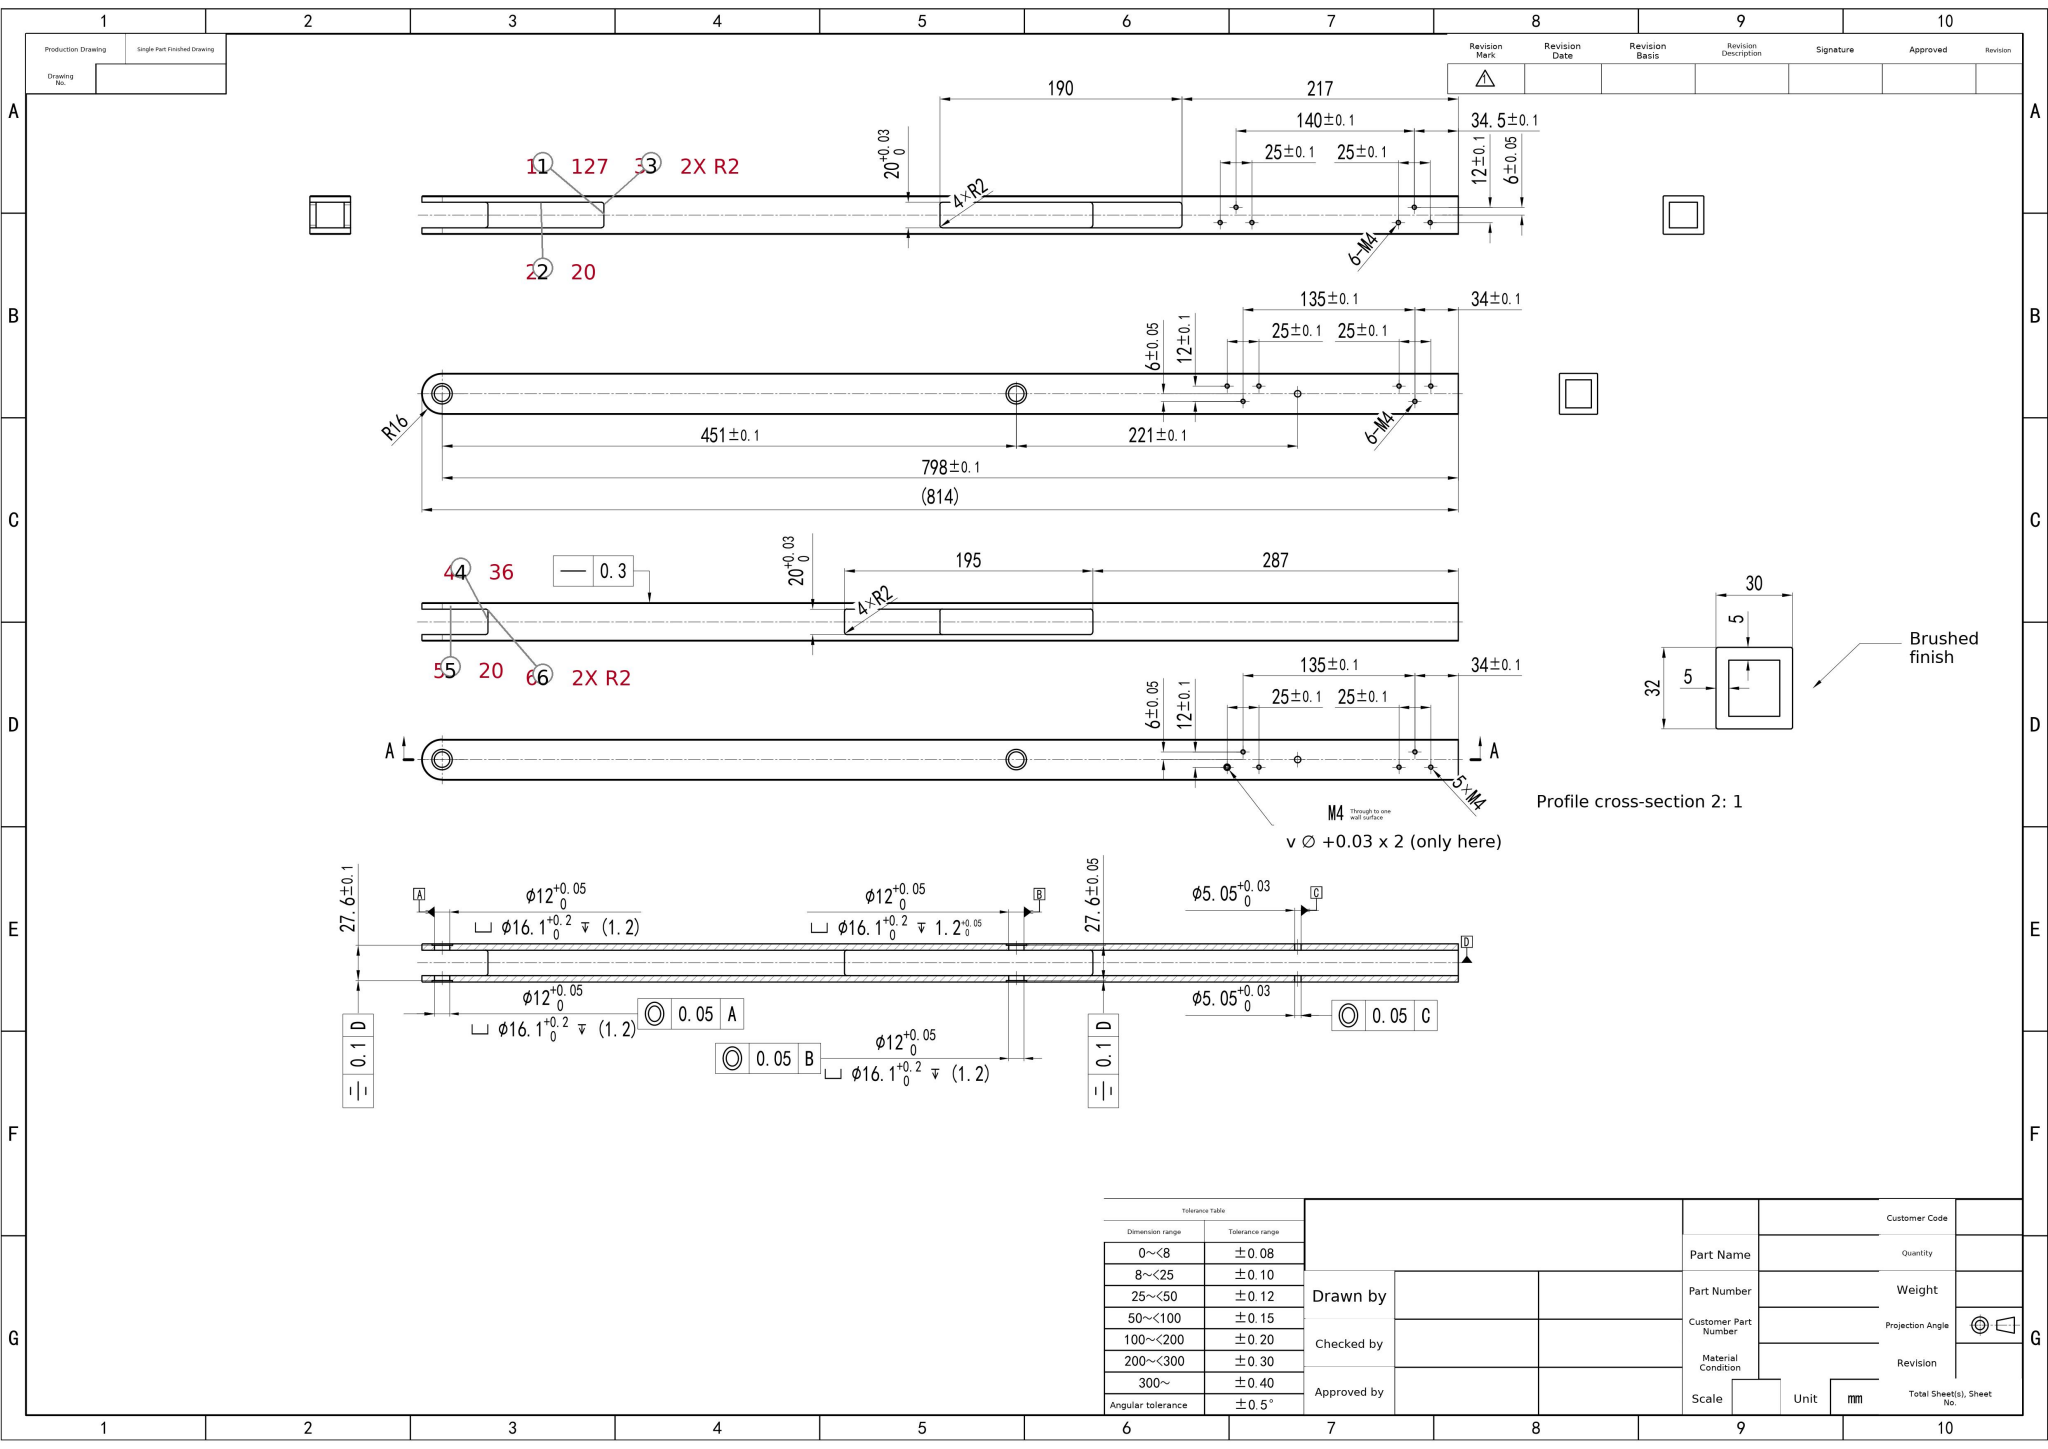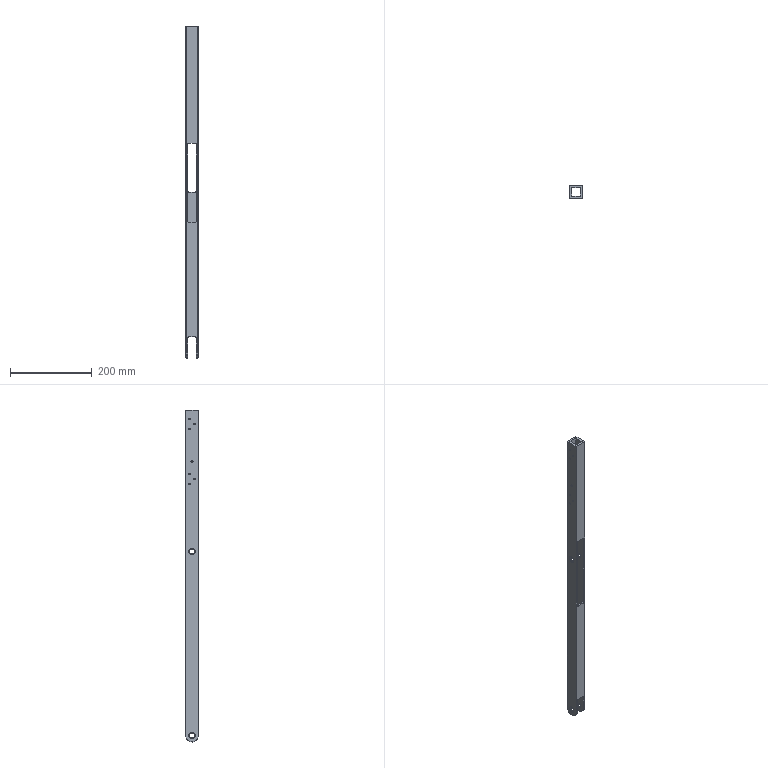Part | SolidWorks | mm | 1 solid | 102 faces | box 30 x 32 x 814 mm | volume 360178 mm3 | cylinder 74 | plane 26 | cone 2 | commonest cylinder face diameters 3.2 x36 4 x12 16.1 x8 12 x8 5.05 x4 32 x4 5 x2